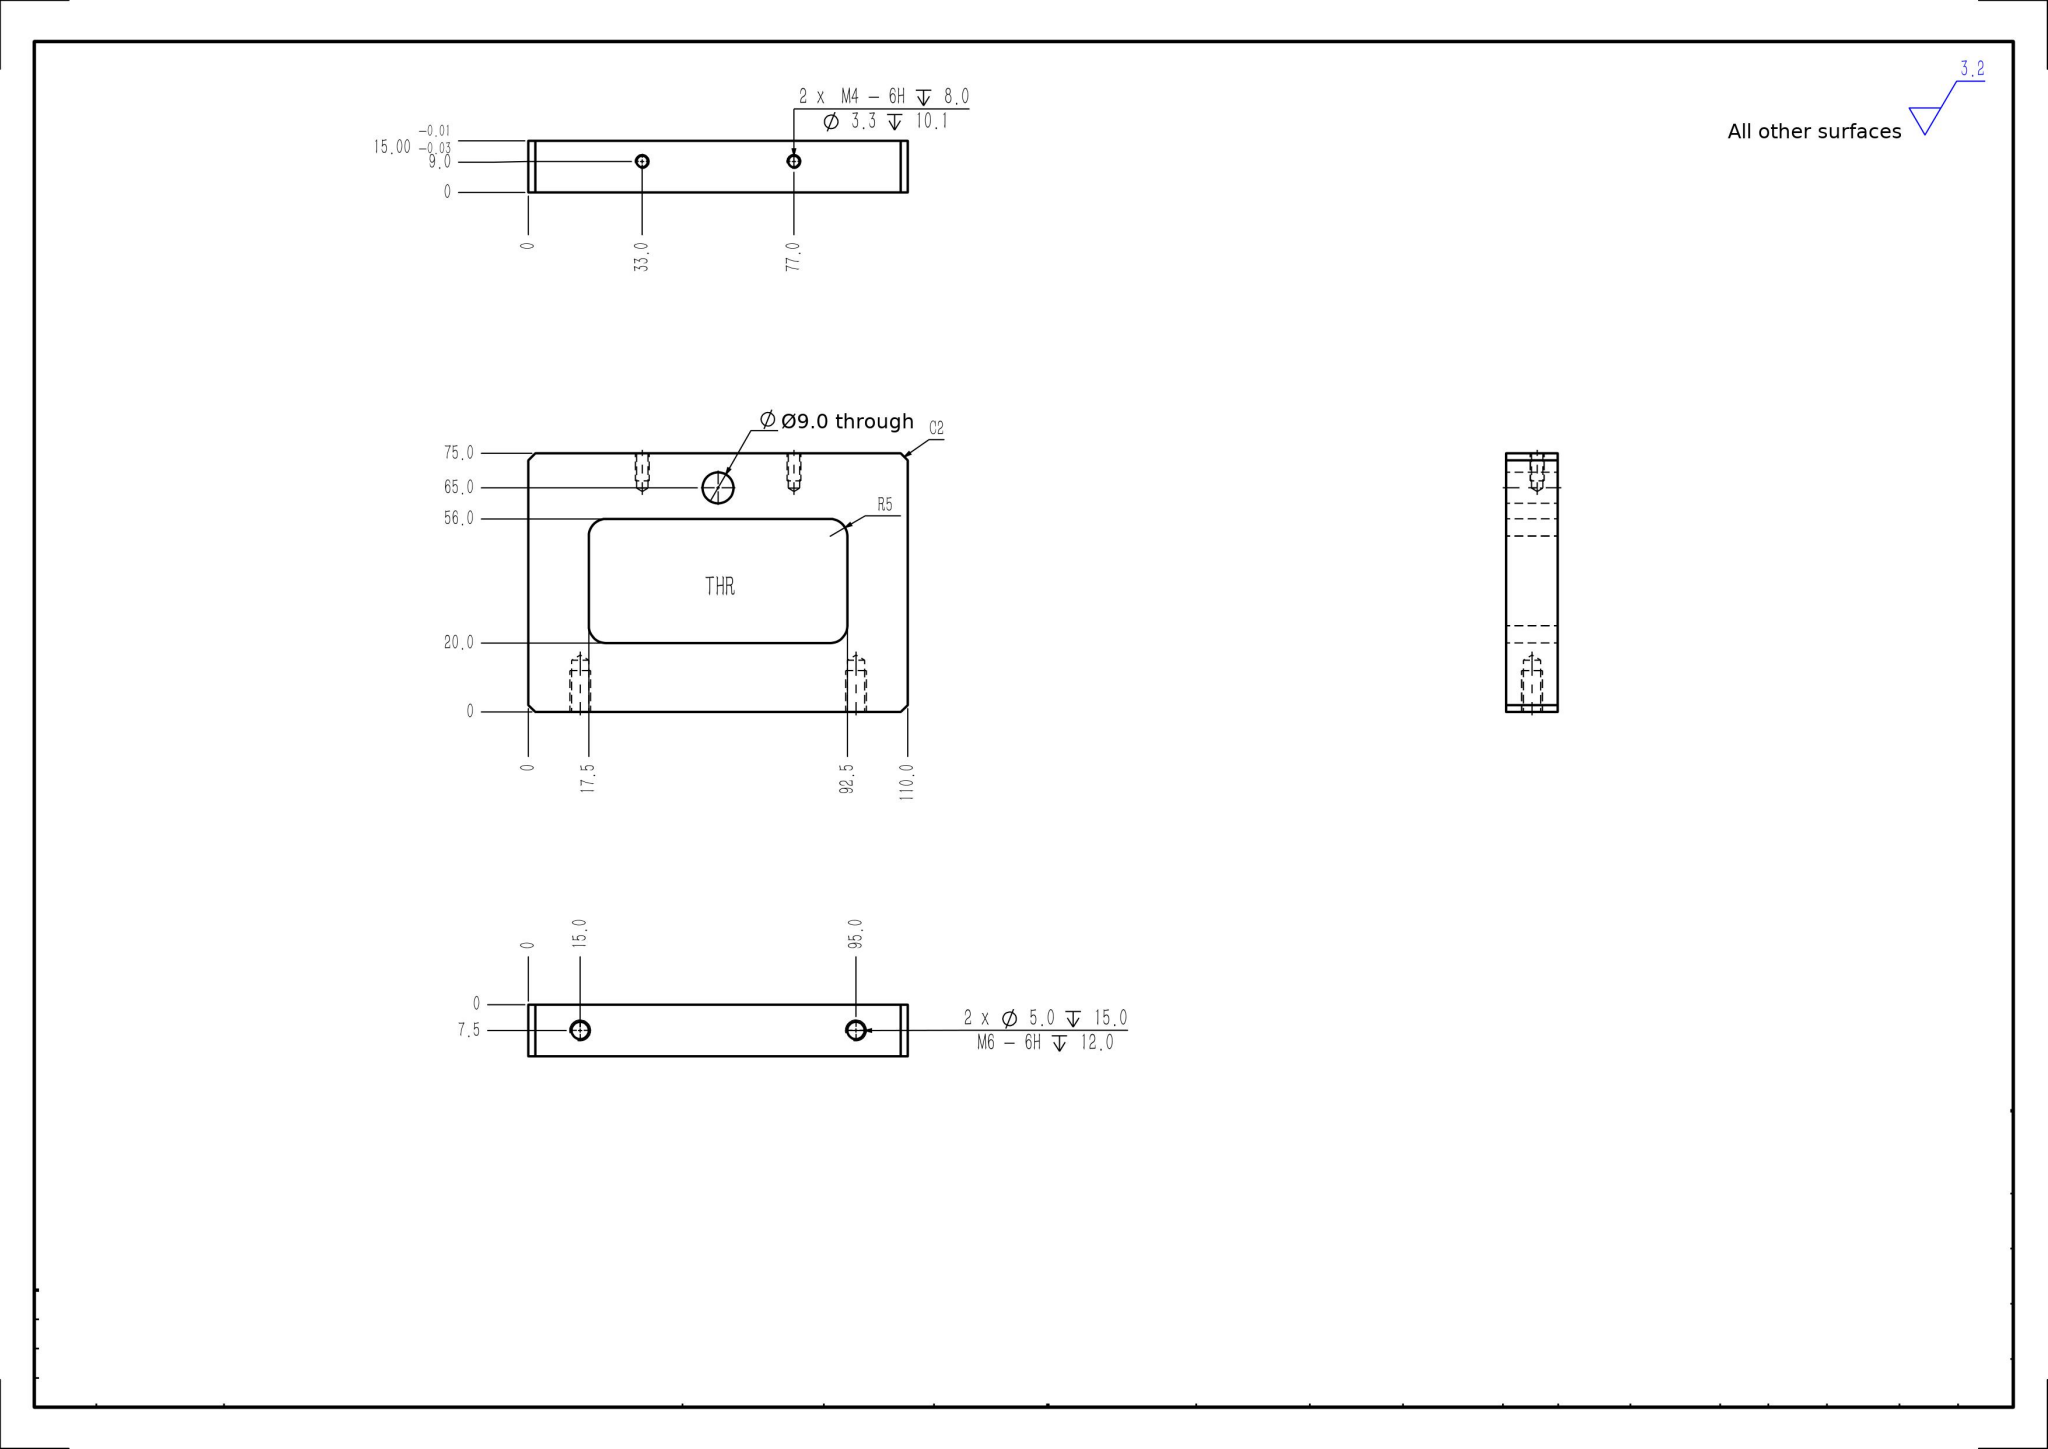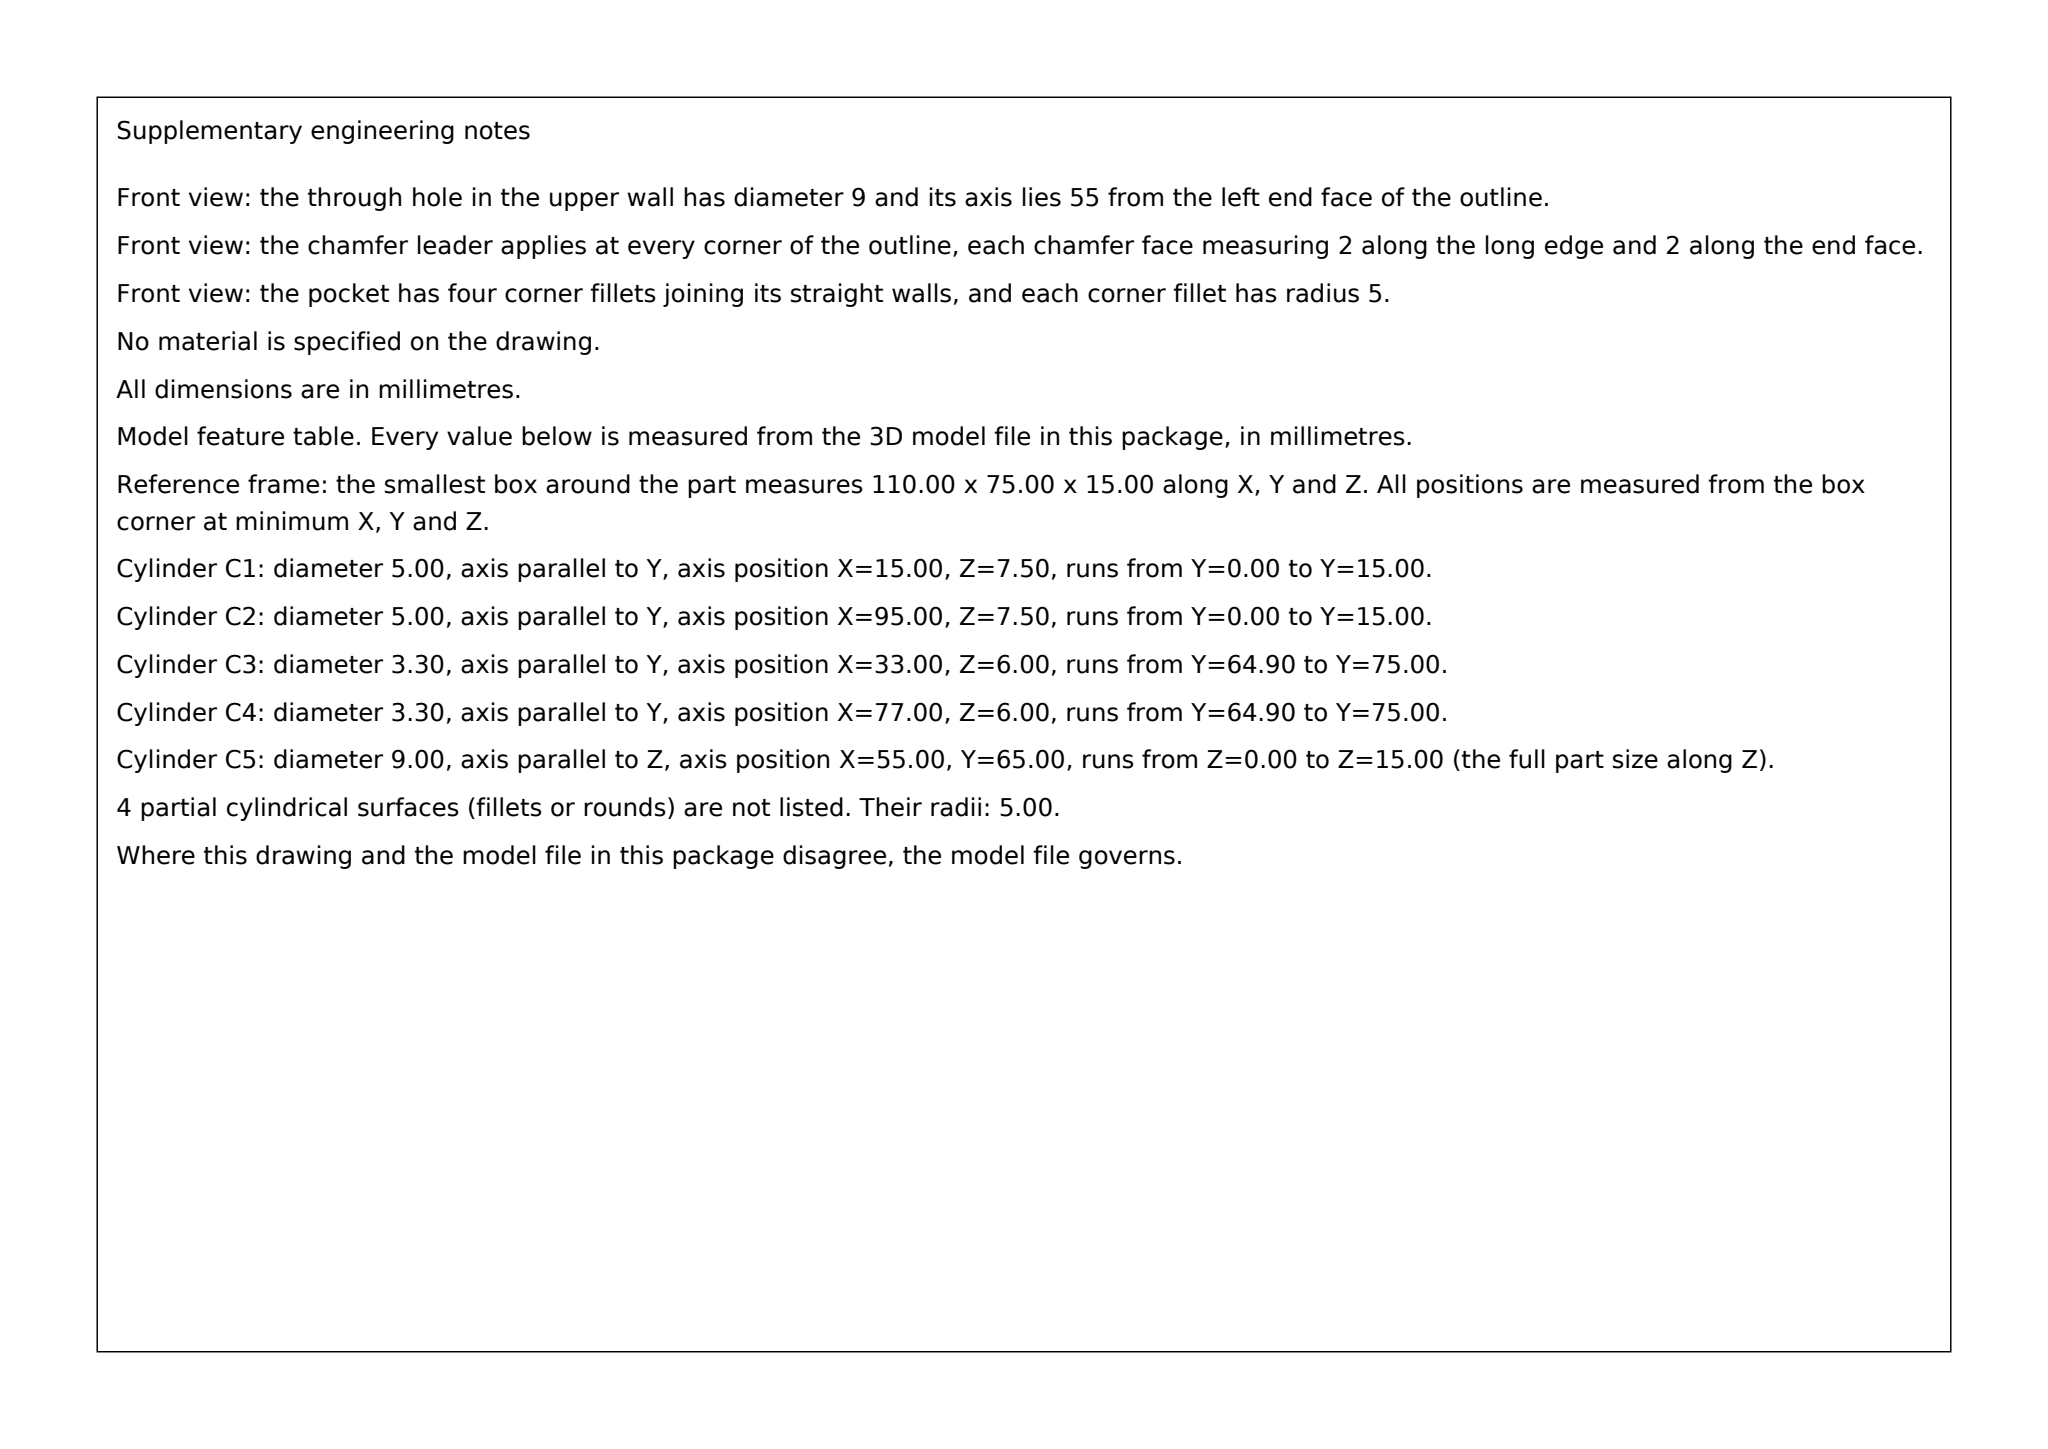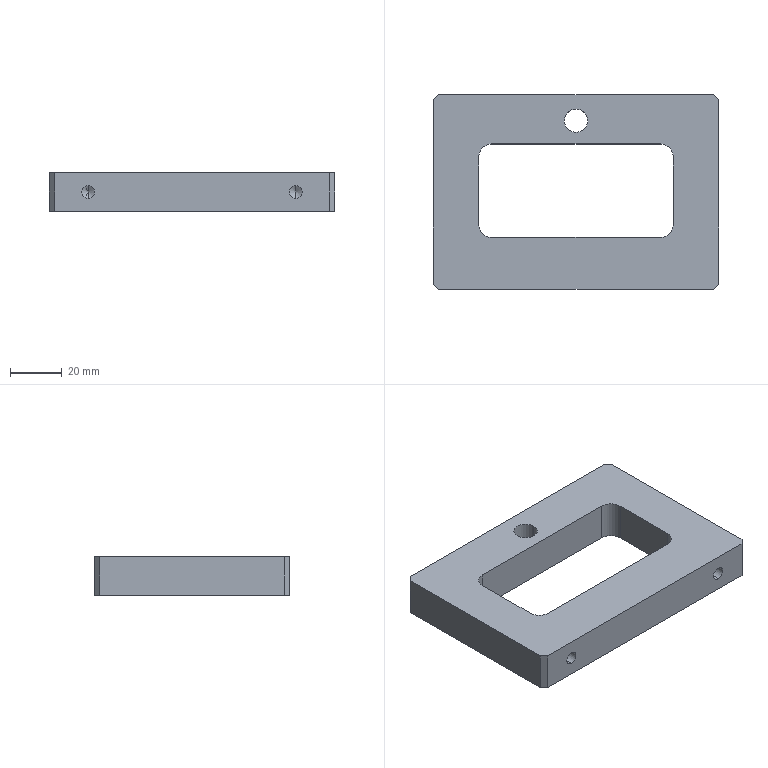Part | SolidWorks | mm | 1 solid | 36 faces | box 110 x 75 x 15 mm | volume 81711 mm3 | cylinder 14 | plane 14 | cone 8 | commonest cylinder face diameters 3.3 x4 5 x4 10 x4 9 x2
Drawing notes:
Ø9.0 THRU, 55.0 FROM LEFT EDGE, 65.0 FROM BOTTOM | from the solid: cylinder dia 9.0 axis z at (x=55.0, y=65.0), length 15.0 = full thk
POCKET 75.0 X 36.0, R5 CORNERS, THRU (15.0 THK) | from the solid: planes x=17.5/92.5, y=20.0/56.0; R5 corner cyls dia10 len 15.0 = bbox z
build123d program:
from build123d import *

# Parameters (mm, degrees)
SKETCH1_W             = 110
SKETCH1_H             = 75
BOSS_EXTRUDE1_DEPTH   = 7.5
M6_TAPPED_HOLE1_D     = 5
M6_TAPPED_HOLE1_DEPTH = 15
M6_TAPPED_HOLE1_TIP   = 1.502
SKETCH8_W             = 75
SKETCH8_H             = 36
CUT_EXTRUDE1_DEPTH    = 95.207
FILLET1_R             = 5
CHAMFER1_SIZE         = 2
SKETCH9_R             = 4.5
CUT_EXTRUDE2_DEPTH    = 95.207
M4_TAPPED_HOLE1_D     = 3.3
M4_TAPPED_HOLE1_DEPTH = 10.1
M4_TAPPED_HOLE1_TIP   = 0.9914


with BuildPart() as part:
    # Sketch1 → Boss-Extrude1 (new, symmetric)
    with BuildSketch(Plane.XY):
        with Locations((0, 37.5)):
            Rectangle(SKETCH1_W, SKETCH1_H)
    extrude(amount=BOSS_EXTRUDE1_DEPTH, both=True)

    # M6 Tapped Hole1
    with Locations(Plane(origin=(0, 0, 0), x_dir=(-1, 0, 0), z_dir=(0, -1, 0))):
        with Locations((-40, 0), (40, 0)):
            Hole(M6_TAPPED_HOLE1_D / 2, depth=M6_TAPPED_HOLE1_DEPTH)
            with Locations((0, 0, -(M6_TAPPED_HOLE1_DEPTH + M6_TAPPED_HOLE1_TIP / 2))):  # 118° drill point
                Cone(0, M6_TAPPED_HOLE1_D / 2, M6_TAPPED_HOLE1_TIP, mode=Mode.SUBTRACT)

    # Sketch8 → Cut-Extrude1 (cut, through all)
    with BuildSketch(Plane(origin=(0, 0, -7.5), x_dir=(-1, 0, 0), z_dir=(0, 0, -1))):
        with Locations((0, 38)):
            Rectangle(SKETCH8_W, SKETCH8_H)
    extrude(amount=-CUT_EXTRUDE1_DEPTH, mode=Mode.SUBTRACT)

    # Fillet1
    fillet1_edges = [part.edges().sort_by_distance(p)[0] for p in [
        (37.5, 20, 0),
        (37.5, 56, 0),
        (-37.5, 56, 0),
        (-37.5, 20, 0),
    ]]
    fillet(fillet1_edges, radius=FILLET1_R)

    # Chamfer1
    chamfer1_edges = [part.edges().sort_by_distance(p)[0] for p in [
        (-55, 75, 0),
        (55, 75, 0),
        (55, 0, 0),
        (-55, 0, 0),
    ]]
    chamfer(chamfer1_edges, length=CHAMFER1_SIZE)

    # Sketch9 → Cut-Extrude2 (cut, through all)
    with BuildSketch(Plane.XY.offset(7.5)):
        with Locations((0, 65)):
            Circle(SKETCH9_R)
    extrude(amount=-CUT_EXTRUDE2_DEPTH, mode=Mode.SUBTRACT)

    # M4 Tapped Hole1
    with Locations(Plane(origin=(0, 75, 0), x_dir=(1, 0, 0), z_dir=(0, 1, 0))):
        with Locations((22, 1.5), (-22, 1.5)):
            Hole(M4_TAPPED_HOLE1_D / 2, depth=M4_TAPPED_HOLE1_DEPTH)
            with Locations((0, 0, -(M4_TAPPED_HOLE1_DEPTH + M4_TAPPED_HOLE1_TIP / 2))):  # 118° drill point
                Cone(0, M4_TAPPED_HOLE1_D / 2, M4_TAPPED_HOLE1_TIP, mode=Mode.SUBTRACT)


solid = part.part